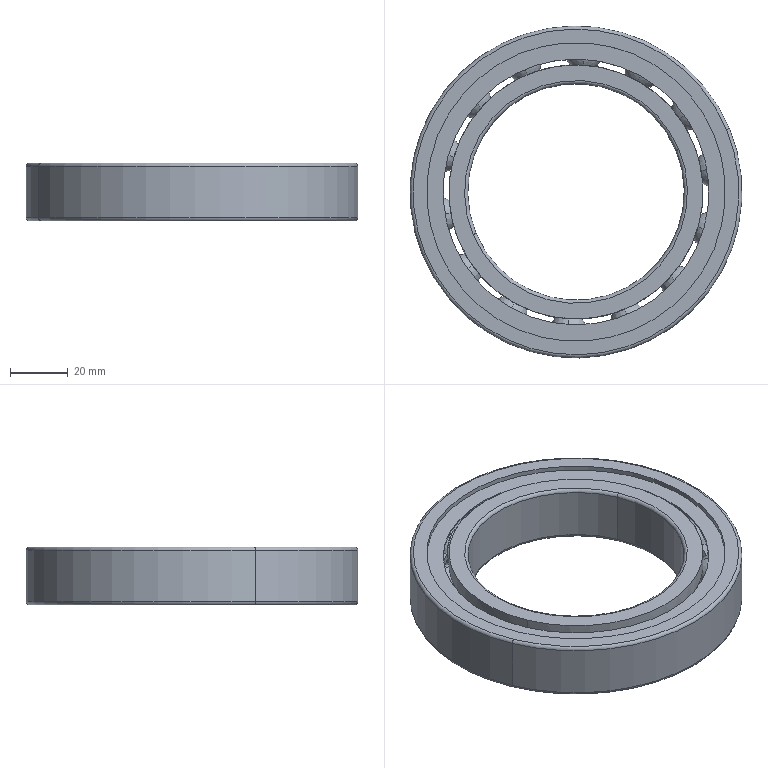Component | SolidWorks | GB_T276-94DeepGrooveBallBearing6015-2RZ-1 | 1 solid | 225 faces | volume 81153 mm3 | sphere 112 | torus 53 | plane 36 | cylinder 24 | commonest cylinder face diameters 103.5 x8 92.06 x4 88 x4 75 x2 115 x2 99.133 x2 92.367 x2 | material GCr4